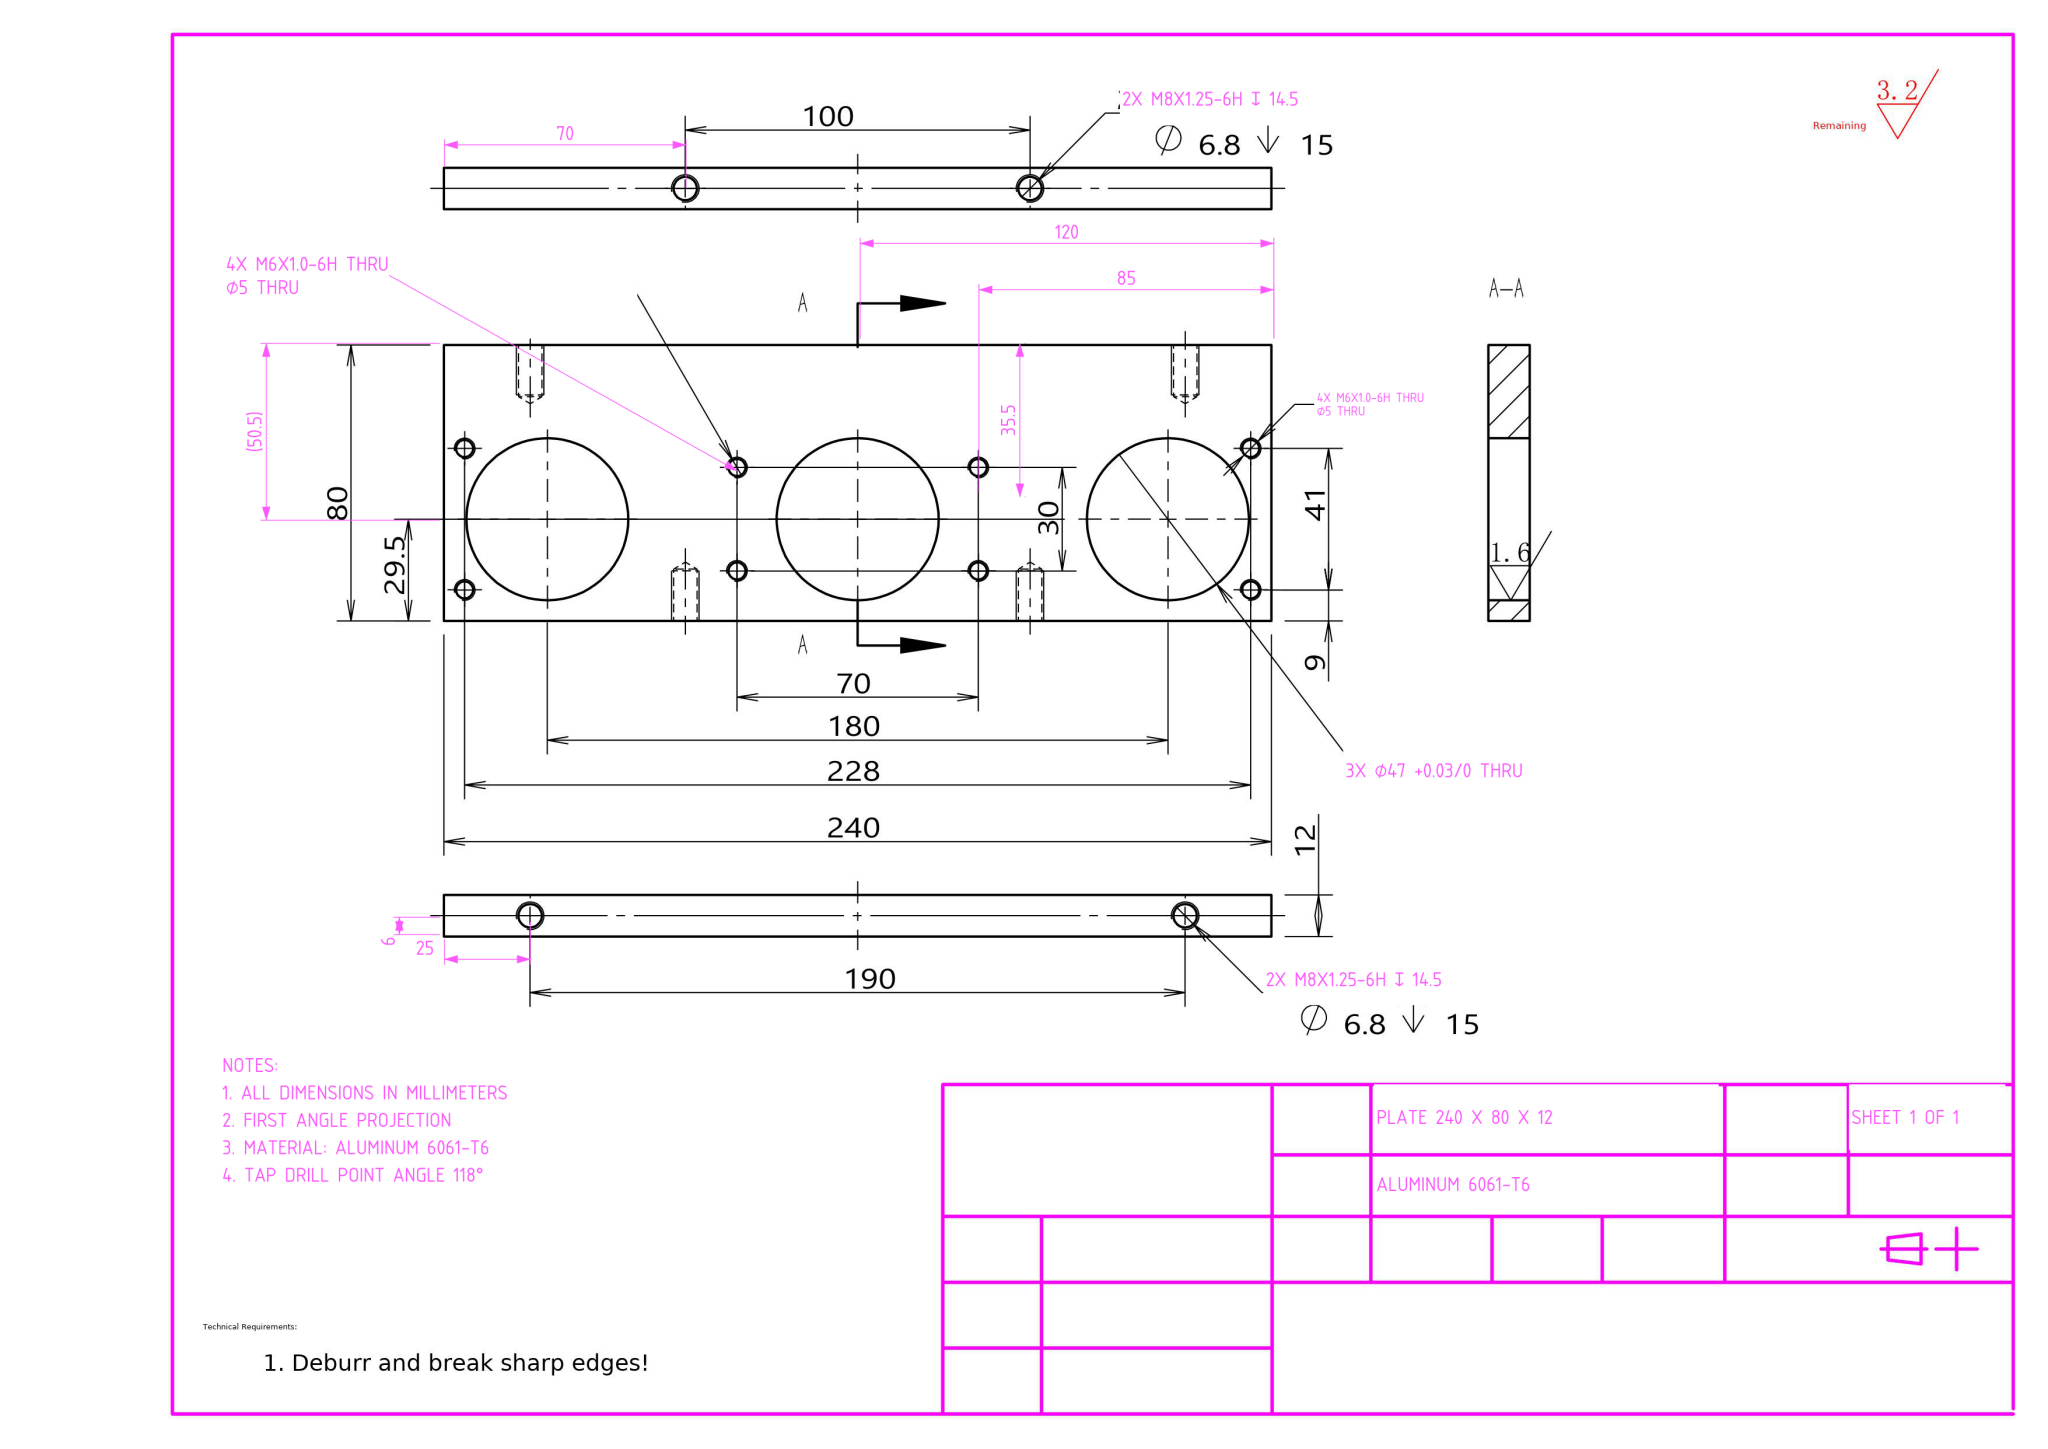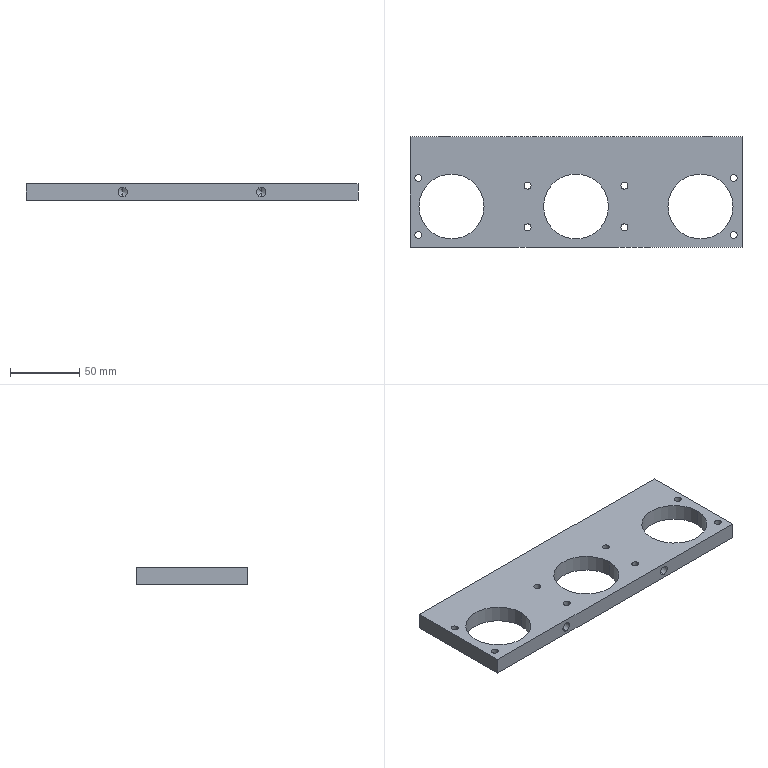Part | NX | mm | 1 solid | 44 faces | box 240 x 80 x 12 mm | volume 163779 mm3 | cylinder 30 | cone 8 | plane 6 | commonest cylinder face diameters 5 x16 6.8 x8 47 x6